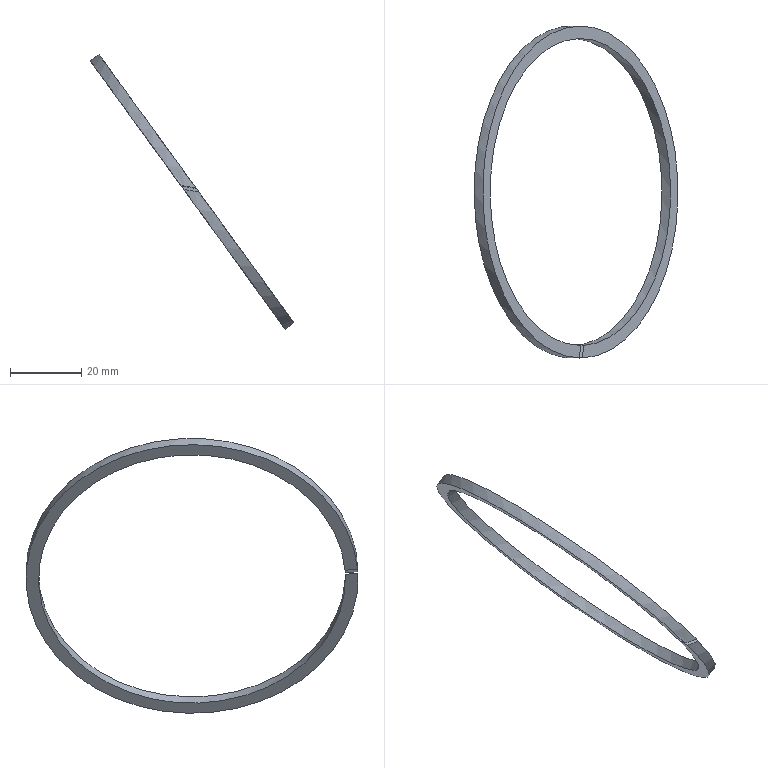Component | NX | PISTON_RING | 1 solid | 6 faces | box 57.09 x 93 x 77 mm | volume 2937 mm3 | plane 4 | cylinder 2 | commonest cylinder face diameters 86 x1 93 x1
STEP:
#1=CARTESIAN_POINT('',(0.,0.,0.));
#2=DIRECTION('',(0.,0.,1.));
#3=DIRECTION('',(1.,0.,0.));
#4=AXIS2_PLACEMENT_3D('',#1,#2,#3);
#5=CARTESIAN_POINT('',(-195.667,-43.,-142.088));
#6=VERTEX_POINT('',#5);
#7=CARTESIAN_POINT('',(-199.858,-42.891,-141.424));
#8=VERTEX_POINT('',#7);
#9=CARTESIAN_POINT('',(-198.06,-0.,-143.899));
#10=DIRECTION('',(-0.1575,-0.0503,-0.9862));
#11=DIRECTION('',(-0.9866,0.0503,0.155));
#12=AXIS2_PLACEMENT_3D('',#9,#10,#11);
#13=ELLIPSE('',#12,60.811,43.);
#14=CARTESIAN_POINT('',(-195.633,-0.,-142.136));
#15=DIRECTION('',(-0.809,0.,-0.5878));
#16=DIRECTION('',(-0.5863,0.07113,0.807));
#17=AXIS2_PLACEMENT_3D('',#14,#15,#16);
#18=CYLINDRICAL_SURFACE('',#17,43.);
#19=CARTESIAN_POINT('',(-1.641,0.));
#20=CARTESIAN_POINT('',(-1.571,3.));
#21=B_SPLINE_CURVE_WITH_KNOTS('',1,(#19,#20),.UNSPECIFIED.,.F.,.F.,(2,2),(4.643,4.712),.PIECEWISE_BEZIER_KNOTS.);
#22=(GEOMETRIC_REPRESENTATION_CONTEXT(2)PARAMETRIC_REPRESENTATION_CONTEXT()REPRESENTATION_CONTEXT('',''));
#23=DEFINITIONAL_REPRESENTATION('',(#21),#22);
#24=PCURVE('',#18,#23);
#25=CARTESIAN_POINT('',(-213.121,-459.397,-118.066));
#26=DIRECTION('',(-0.1575,-0.0503,-0.9862));
#27=DIRECTION('',(-0.9866,0.0503,0.155));
#28=AXIS2_PLACEMENT_3D('',#25,#26,#27);
#29=PLANE('',#28);
#30=CARTESIAN_POINT('',(4.243,460.35));
#31=DIRECTION('',(1.,0.));
#32=AXIS2_PLACEMENT_2D('',#30,#31);
#33=ELLIPSE('',#32,60.811,43.);
#34=(GEOMETRIC_REPRESENTATION_CONTEXT(2)PARAMETRIC_REPRESENTATION_CONTEXT()REPRESENTATION_CONTEXT('',''));
#35=DEFINITIONAL_REPRESENTATION('',(#33),#34);
#36=PCURVE('',#29,#35);
#37=SURFACE_CURVE('',#13,(#24,#36),.PCURVE_S1.);
#38=EDGE_CURVE('',#6,#8,#37,.T.);
#39=ORIENTED_EDGE('',*,*,#38,.F.);
#40=CARTESIAN_POINT('',(-194.833,-42.978,-143.236));
#41=VERTEX_POINT('',#40);
#42=CARTESIAN_POINT('',(-195.633,-0.,-142.136));
#43=DIRECTION('',(0.809,0.,0.5878));
#44=DIRECTION('',(0.5863,-0.07113,-0.807));
#45=AXIS2_PLACEMENT_3D('',#42,#43,#44);
#46=CIRCLE('',#45,43.);
#47=CARTESIAN_POINT('',(9.425,-0.));
#48=DIRECTION('',(-1.,0.));
#49=VECTOR('',#48,1.);
#50=LINE('',#47,#49);
#51=(GEOMETRIC_REPRESENTATION_CONTEXT(2)PARAMETRIC_REPRESENTATION_CONTEXT()REPRESENTATION_CONTEXT('',''));
#52=DEFINITIONAL_REPRESENTATION('',(#50),#51);
#53=PCURVE('',#18,#52);
#54=CARTESIAN_POINT('',(-195.633,-0.,-142.136));
#55=DIRECTION('',(0.809,0.,0.5878));
#56=DIRECTION('',(0.5863,-0.07113,-0.807));
#57=AXIS2_PLACEMENT_3D('',#54,#55,#56);
#58=PLANE('',#57);
#59=CARTESIAN_POINT('',(0.,0.));
#60=DIRECTION('',(1.,0.));
#61=AXIS2_PLACEMENT_2D('',#59,#60);
#62=CIRCLE('',#61,43.);
#63=(GEOMETRIC_REPRESENTATION_CONTEXT(2)PARAMETRIC_REPRESENTATION_CONTEXT()REPRESENTATION_CONTEXT('',''));
#64=DEFINITIONAL_REPRESENTATION('',(#62),#63);
#65=PCURVE('',#58,#64);
#66=SURFACE_CURVE('',#46,(#53,#65),.PCURVE_S1.);
#67=EDGE_CURVE('',#41,#6,#66,.T.);
#68=ORIENTED_EDGE('',*,*,#67,.F.);
#69=CARTESIAN_POINT('',(-199.027,-42.968,-142.567));
#70=VERTEX_POINT('',#69);
#71=CARTESIAN_POINT('',(-199.204,-0.,-144.73));
#72=DIRECTION('',(0.1575,0.0503,0.9862));
#73=DIRECTION('',(-0.9866,0.0503,0.155));
#74=AXIS2_PLACEMENT_3D('',#71,#72,#73);
#75=ELLIPSE('',#74,60.811,43.);
#76=CARTESIAN_POINT('',(4.679,3.));
#77=CARTESIAN_POINT('',(4.61,0.));
#78=B_SPLINE_CURVE_WITH_KNOTS('',1,(#76,#77),.UNSPECIFIED.,.F.,.F.,(2,2),(1.604,1.674),.PIECEWISE_BEZIER_KNOTS.);
#79=(GEOMETRIC_REPRESENTATION_CONTEXT(2)PARAMETRIC_REPRESENTATION_CONTEXT()REPRESENTATION_CONTEXT('',''));
#80=DEFINITIONAL_REPRESENTATION('',(#78),#79);
#81=PCURVE('',#18,#80);
#82=CARTESIAN_POINT('',(-216.477,-459.285,-118.549));
#83=DIRECTION('',(0.1575,0.0503,0.9862));
#84=DIRECTION('',(0.9866,-0.0503,-0.155));
#85=AXIS2_PLACEMENT_3D('',#82,#83,#84);
#86=PLANE('',#85);
#87=CARTESIAN_POINT('',(-2.,460.35));
#88=DIRECTION('',(-1.,0.));
#89=AXIS2_PLACEMENT_2D('',#87,#88);
#90=ELLIPSE('',#89,60.811,43.);
#91=(GEOMETRIC_REPRESENTATION_CONTEXT(2)PARAMETRIC_REPRESENTATION_CONTEXT()REPRESENTATION_CONTEXT('',''));
#92=DEFINITIONAL_REPRESENTATION('',(#90),#91);
#93=PCURVE('',#86,#92);
#94=SURFACE_CURVE('',#75,(#81,#93),.PCURVE_S1.);
#95=EDGE_CURVE('',#70,#41,#94,.T.);
#96=ORIENTED_EDGE('',*,*,#95,.F.);
#97=CARTESIAN_POINT('',(-198.06,-0.,-143.899));
#98=DIRECTION('',(0.809,0.,0.5878));
#99=DIRECTION('',(0.5863,-0.07113,-0.807));
#100=AXIS2_PLACEMENT_3D('',#97,#98,#99);
#101=CIRCLE('',#100,43.);
#102=CARTESIAN_POINT('',(9.425,3.));
#103=DIRECTION('',(-1.,0.));
#104=VECTOR('',#103,1.);
#105=LINE('',#102,#104);
#106=(GEOMETRIC_REPRESENTATION_CONTEXT(2)PARAMETRIC_REPRESENTATION_CONTEXT()REPRESENTATION_CONTEXT('',''));
#107=DEFINITIONAL_REPRESENTATION('',(#105),#106);
#108=PCURVE('',#18,#107);
#109=CARTESIAN_POINT('',(-198.06,-0.,-143.899));
#110=DIRECTION('',(0.809,0.,0.5878));
#111=DIRECTION('',(0.5863,-0.07113,-0.807));
#112=AXIS2_PLACEMENT_3D('',#109,#110,#111);
#113=PLANE('',#112);
#114=CARTESIAN_POINT('',(0.,0.));
#115=DIRECTION('',(1.,0.));
#116=AXIS2_PLACEMENT_2D('',#114,#115);
#117=CIRCLE('',#116,43.);
#118=(GEOMETRIC_REPRESENTATION_CONTEXT(2)PARAMETRIC_REPRESENTATION_CONTEXT()REPRESENTATION_CONTEXT('',''));
#119=DEFINITIONAL_REPRESENTATION('',(#117),#118);
#120=PCURVE('',#113,#119);
#121=SURFACE_CURVE('',#101,(#108,#120),.PCURVE_S1.);
#122=EDGE_CURVE('',#70,#8,#121,.T.);
#123=ORIENTED_EDGE('',*,*,#122,.T.);
#124=EDGE_LOOP('',(#39,#68,#96,#123));
#125=FACE_BOUND('',#124,.F.);
#126=ADVANCED_FACE('',(#125),#18,.F.);
#127=CARTESIAN_POINT('',(-194.98,-46.487,-143.034));
#128=VERTEX_POINT('',#127);
#129=CARTESIAN_POINT('',(-195.814,-46.499,-141.886));
#130=VERTEX_POINT('',#129);
#131=CARTESIAN_POINT('',(-195.633,-0.,-142.136));
#132=DIRECTION('',(0.809,0.,0.5878));
#133=DIRECTION('',(0.5863,-0.07113,-0.807));
#134=AXIS2_PLACEMENT_3D('',#131,#132,#133);
#135=CIRCLE('',#134,46.5);
#136=CARTESIAN_POINT('',(0.,0.));
#137=DIRECTION('',(1.,0.));
#138=AXIS2_PLACEMENT_2D('',#136,#137);
#139=CIRCLE('',#138,46.5);
#140=(GEOMETRIC_REPRESENTATION_CONTEXT(2)PARAMETRIC_REPRESENTATION_CONTEXT()REPRESENTATION_CONTEXT('',''));
#141=DEFINITIONAL_REPRESENTATION('',(#139),#140);
#142=PCURVE('',#58,#141);
#143=CARTESIAN_POINT('',(-195.633,-0.,-142.136));
#144=DIRECTION('',(-0.809,0.,-0.5878));
#145=DIRECTION('',(-0.5863,0.07113,0.807));
#146=AXIS2_PLACEMENT_3D('',#143,#144,#145);
#147=CYLINDRICAL_SURFACE('',#146,46.5);
#148=CARTESIAN_POINT('',(9.425,-0.));
#149=DIRECTION('',(-1.,0.));
#150=VECTOR('',#149,1.);
#151=LINE('',#148,#150);
#152=(GEOMETRIC_REPRESENTATION_CONTEXT(2)PARAMETRIC_REPRESENTATION_CONTEXT()REPRESENTATION_CONTEXT('',''));
#153=DEFINITIONAL_REPRESENTATION('',(#151),#152);
#154=PCURVE('',#147,#153);
#155=SURFACE_CURVE('',#135,(#142,#154),.PCURVE_S1.);
#156=EDGE_CURVE('',#128,#130,#155,.T.);
#157=ORIENTED_EDGE('',*,*,#156,.T.);
#158=CARTESIAN_POINT('',(-213.121,-459.397,-118.066));
#159=DIRECTION('',(0.04181,0.9975,-0.05754));
#160=VECTOR('',#159,1.);
#161=LINE('',#158,#160);
#162=CARTESIAN_POINT('',(3.,-460.35));
#163=DIRECTION('',(0.,1.));
#164=VECTOR('',#163,1.);
#165=LINE('',#162,#164);
#166=(GEOMETRIC_REPRESENTATION_CONTEXT(2)PARAMETRIC_REPRESENTATION_CONTEXT()REPRESENTATION_CONTEXT('',''));
#167=DEFINITIONAL_REPRESENTATION('',(#165),#166);
#168=PCURVE('',#58,#167);
#169=CARTESIAN_POINT('',(0.,0.));
#170=DIRECTION('',(-0.,1.));
#171=VECTOR('',#170,1.);
#172=LINE('',#169,#171);
#173=(GEOMETRIC_REPRESENTATION_CONTEXT(2)PARAMETRIC_REPRESENTATION_CONTEXT()REPRESENTATION_CONTEXT('',''));
#174=DEFINITIONAL_REPRESENTATION('',(#172),#173);
#175=PCURVE('',#29,#174);
#176=SURFACE_CURVE('',#161,(#168,#175),.PCURVE_S1.);
#177=EDGE_CURVE('',#130,#6,#176,.T.);
#178=ORIENTED_EDGE('',*,*,#177,.T.);
#179=ORIENTED_EDGE('',*,*,#67,.F.);
#180=CARTESIAN_POINT('',(-212.291,-459.498,-119.207));
#181=DIRECTION('',(0.04181,0.9975,-0.05754));
#182=VECTOR('',#181,1.);
#183=LINE('',#180,#182);
#184=CARTESIAN_POINT('',(4.414,-460.35));
#185=DIRECTION('',(0.,1.));
#186=VECTOR('',#185,1.);
#187=LINE('',#184,#186);
#188=(GEOMETRIC_REPRESENTATION_CONTEXT(2)PARAMETRIC_REPRESENTATION_CONTEXT()REPRESENTATION_CONTEXT('',''));
#189=DEFINITIONAL_REPRESENTATION('',(#187),#188);
#190=PCURVE('',#58,#189);
#191=CARTESIAN_POINT('',(4.243,0.));
#192=DIRECTION('',(0.,1.));
#193=VECTOR('',#192,1.);
#194=LINE('',#191,#193);
#195=(GEOMETRIC_REPRESENTATION_CONTEXT(2)PARAMETRIC_REPRESENTATION_CONTEXT()REPRESENTATION_CONTEXT('',''));
#196=DEFINITIONAL_REPRESENTATION('',(#194),#195);
#197=PCURVE('',#86,#196);
#198=SURFACE_CURVE('',#183,(#190,#197),.PCURVE_S1.);
#199=EDGE_CURVE('',#128,#41,#198,.T.);
#200=ORIENTED_EDGE('',*,*,#199,.F.);
#201=EDGE_LOOP('',(#157,#178,#179,#200));
#202=FACE_BOUND('',#201,.T.);
#203=ADVANCED_FACE('',(#202),#58,.T.);
#204=ORIENTED_EDGE('',*,*,#156,.F.);
#205=CARTESIAN_POINT('',(-199.174,-46.461,-142.366));
#206=VERTEX_POINT('',#205);
#207=CARTESIAN_POINT('',(-199.204,-0.,-144.73));
#208=DIRECTION('',(-0.1575,-0.0503,-0.9862));
#209=DIRECTION('',(-0.9866,0.0503,0.155));
#210=AXIS2_PLACEMENT_3D('',#207,#208,#209);
#211=ELLIPSE('',#210,65.761,46.5);
#212=CARTESIAN_POINT('',(4.617,0.));
#213=CARTESIAN_POINT('',(4.682,3.));
#214=B_SPLINE_CURVE_WITH_KNOTS('',1,(#212,#213),.UNSPECIFIED.,.F.,.F.,(2,2),(4.617,4.682),.PIECEWISE_BEZIER_KNOTS.);
#215=(GEOMETRIC_REPRESENTATION_CONTEXT(2)PARAMETRIC_REPRESENTATION_CONTEXT()REPRESENTATION_CONTEXT('',''));
#216=DEFINITIONAL_REPRESENTATION('',(#214),#215);
#217=PCURVE('',#147,#216);
#218=CARTESIAN_POINT('',(-67.761,460.35));
#219=CARTESIAN_POINT('',(-67.761,540.89));
#220=CARTESIAN_POINT('',(30.88,500.62));
#221=CARTESIAN_POINT('',(129.522,460.35));
#222=CARTESIAN_POINT('',(30.88,420.08));
#223=CARTESIAN_POINT('',(-67.761,379.81));
#224=CARTESIAN_POINT('',(-67.761,460.35));
#225=(BOUNDED_CURVE()B_SPLINE_CURVE(2,(#218,#219,#220,#221,#222,#223,#224),.UNSPECIFIED.,.T.,.F.)B_SPLINE_CURVE_WITH_KNOTS((1,2,2,2,2,1),(-2.094,0.,2.094,4.189,6.283,8.378),.UNSPECIFIED.)CURVE()GEOMETRIC_REPRESENTATION_ITEM()RATIONAL_B_SPLINE_CURVE((1.,0.5,1.,0.5,1.,0.5,1.))REPRESENTATION_ITEM(''));
#226=(GEOMETRIC_REPRESENTATION_CONTEXT(2)PARAMETRIC_REPRESENTATION_CONTEXT()REPRESENTATION_CONTEXT('',''));
#227=DEFINITIONAL_REPRESENTATION('',(#225),#226);
#228=PCURVE('',#86,#227);
#229=SURFACE_CURVE('',#211,(#217,#228),.PCURVE_S1.);
#230=EDGE_CURVE('',#128,#206,#229,.T.);
#231=ORIENTED_EDGE('',*,*,#230,.T.);
#232=CARTESIAN_POINT('',(-200.004,-46.382,-141.223));
#233=VERTEX_POINT('',#232);
#234=CARTESIAN_POINT('',(-198.06,-0.,-143.899));
#235=DIRECTION('',(0.809,0.,0.5878));
#236=DIRECTION('',(0.5863,-0.07113,-0.807));
#237=AXIS2_PLACEMENT_3D('',#234,#235,#236);
#238=CIRCLE('',#237,46.5);
#239=CARTESIAN_POINT('',(9.425,3.));
#240=DIRECTION('',(-1.,0.));
#241=VECTOR('',#240,1.);
#242=LINE('',#239,#241);
#243=(GEOMETRIC_REPRESENTATION_CONTEXT(2)PARAMETRIC_REPRESENTATION_CONTEXT()REPRESENTATION_CONTEXT('',''));
#244=DEFINITIONAL_REPRESENTATION('',(#242),#243);
#245=PCURVE('',#147,#244);
#246=CARTESIAN_POINT('',(0.,0.));
#247=DIRECTION('',(1.,0.));
#248=AXIS2_PLACEMENT_2D('',#246,#247);
#249=CIRCLE('',#248,46.5);
#250=(GEOMETRIC_REPRESENTATION_CONTEXT(2)PARAMETRIC_REPRESENTATION_CONTEXT()REPRESENTATION_CONTEXT('',''));
#251=DEFINITIONAL_REPRESENTATION('',(#249),#250);
#252=PCURVE('',#113,#251);
#253=SURFACE_CURVE('',#238,(#245,#252),.PCURVE_S1.);
#254=EDGE_CURVE('',#206,#233,#253,.T.);
#255=ORIENTED_EDGE('',*,*,#254,.T.);
#256=CARTESIAN_POINT('',(-198.06,-0.,-143.899));
#257=DIRECTION('',(0.1575,0.0503,0.9862));
#258=DIRECTION('',(-0.9866,0.0503,0.155));
#259=AXIS2_PLACEMENT_3D('',#256,#257,#258);
#260=ELLIPSE('',#259,65.761,46.5);
#261=CARTESIAN_POINT('',(-1.571,3.));
#262=CARTESIAN_POINT('',(-1.635,0.));
#263=B_SPLINE_CURVE_WITH_KNOTS('',1,(#261,#262),.UNSPECIFIED.,.F.,.F.,(2,2),(1.571,1.635),.PIECEWISE_BEZIER_KNOTS.);
#264=(GEOMETRIC_REPRESENTATION_CONTEXT(2)PARAMETRIC_REPRESENTATION_CONTEXT()REPRESENTATION_CONTEXT('',''));
#265=DEFINITIONAL_REPRESENTATION('',(#263),#264);
#266=PCURVE('',#147,#265);
#267=CARTESIAN_POINT('',(70.004,460.35));
#268=CARTESIAN_POINT('',(70.004,379.81));
#269=CARTESIAN_POINT('',(-28.638,420.08));
#270=CARTESIAN_POINT('',(-127.279,460.35));
#271=CARTESIAN_POINT('',(-28.638,500.62));
#272=CARTESIAN_POINT('',(70.004,540.89));
#273=CARTESIAN_POINT('',(70.004,460.35));
#274=(BOUNDED_CURVE()B_SPLINE_CURVE(2,(#267,#268,#269,#270,#271,#272,#273),.UNSPECIFIED.,.T.,.F.)B_SPLINE_CURVE_WITH_KNOTS((1,2,2,2,2,1),(-2.094,0.,2.094,4.189,6.283,8.378),.UNSPECIFIED.)CURVE()GEOMETRIC_REPRESENTATION_ITEM()RATIONAL_B_SPLINE_CURVE((1.,0.5,1.,0.5,1.,0.5,1.))REPRESENTATION_ITEM(''));
#275=(GEOMETRIC_REPRESENTATION_CONTEXT(2)PARAMETRIC_REPRESENTATION_CONTEXT()REPRESENTATION_CONTEXT('',''));
#276=DEFINITIONAL_REPRESENTATION('',(#274),#275);
#277=PCURVE('',#29,#276);
#278=SURFACE_CURVE('',#260,(#266,#277),.PCURVE_S1.);
#279=EDGE_CURVE('',#233,#130,#278,.T.);
#280=ORIENTED_EDGE('',*,*,#279,.T.);
#281=EDGE_LOOP('',(#204,#231,#255,#280));
#282=FACE_BOUND('',#281,.T.);
#283=ADVANCED_FACE('',(#282),#147,.T.);
#284=ORIENTED_EDGE('',*,*,#254,.F.);
#285=CARTESIAN_POINT('',(-216.477,-459.285,-118.549));
#286=DIRECTION('',(0.04181,0.9975,-0.05754));
#287=VECTOR('',#286,1.);
#288=LINE('',#285,#287);
#289=CARTESIAN_POINT('',(1.414,-460.35));
#290=DIRECTION('',(0.,1.));
#291=VECTOR('',#290,1.);
#292=LINE('',#289,#291);
#293=(GEOMETRIC_REPRESENTATION_CONTEXT(2)PARAMETRIC_REPRESENTATION_CONTEXT()REPRESENTATION_CONTEXT('',''));
#294=DEFINITIONAL_REPRESENTATION('',(#292),#293);
#295=PCURVE('',#113,#294);
#296=CARTESIAN_POINT('',(0.,0.));
#297=DIRECTION('',(0.,1.));
#298=VECTOR('',#297,1.);
#299=LINE('',#296,#298);
#300=(GEOMETRIC_REPRESENTATION_CONTEXT(2)PARAMETRIC_REPRESENTATION_CONTEXT()REPRESENTATION_CONTEXT('',''));
#301=DEFINITIONAL_REPRESENTATION('',(#299),#300);
#302=PCURVE('',#86,#301);
#303=SURFACE_CURVE('',#288,(#295,#302),.PCURVE_S1.);
#304=EDGE_CURVE('',#206,#70,#303,.T.);
#305=ORIENTED_EDGE('',*,*,#304,.T.);
#306=ORIENTED_EDGE('',*,*,#122,.T.);
#307=CARTESIAN_POINT('',(-217.307,-459.184,-117.408));
#308=DIRECTION('',(0.04181,0.9975,-0.05754));
#309=VECTOR('',#308,1.);
#310=LINE('',#307,#309);
#311=CARTESIAN_POINT('',(-0.,-460.35));
#312=DIRECTION('',(0.,1.));
#313=VECTOR('',#312,1.);
#314=LINE('',#311,#313);
#315=(GEOMETRIC_REPRESENTATION_CONTEXT(2)PARAMETRIC_REPRESENTATION_CONTEXT()REPRESENTATION_CONTEXT('',''));
#316=DEFINITIONAL_REPRESENTATION('',(#314),#315);
#317=PCURVE('',#113,#316);
#318=CARTESIAN_POINT('',(4.243,0.));
#319=DIRECTION('',(-0.,1.));
#320=VECTOR('',#319,1.);
#321=LINE('',#318,#320);
#322=(GEOMETRIC_REPRESENTATION_CONTEXT(2)PARAMETRIC_REPRESENTATION_CONTEXT()REPRESENTATION_CONTEXT('',''));
#323=DEFINITIONAL_REPRESENTATION('',(#321),#322);
#324=PCURVE('',#29,#323);
#325=SURFACE_CURVE('',#310,(#317,#324),.PCURVE_S1.);
#326=EDGE_CURVE('',#233,#8,#325,.T.);
#327=ORIENTED_EDGE('',*,*,#326,.F.);
#328=EDGE_LOOP('',(#284,#305,#306,#327));
#329=FACE_BOUND('',#328,.T.);
#330=ADVANCED_FACE('',(#329),#113,.F.);
#331=ORIENTED_EDGE('',*,*,#177,.F.);
#332=ORIENTED_EDGE('',*,*,#279,.F.);
#333=ORIENTED_EDGE('',*,*,#326,.T.);
#334=ORIENTED_EDGE('',*,*,#38,.F.);
#335=EDGE_LOOP('',(#331,#332,#333,#334));
#336=FACE_BOUND('',#335,.T.);
#337=ADVANCED_FACE('',(#336),#29,.T.);
#338=ORIENTED_EDGE('',*,*,#304,.F.);
#339=ORIENTED_EDGE('',*,*,#230,.F.);
#340=ORIENTED_EDGE('',*,*,#199,.T.);
#341=ORIENTED_EDGE('',*,*,#95,.F.);
#342=EDGE_LOOP('',(#338,#339,#340,#341));
#343=FACE_BOUND('',#342,.T.);
#344=ADVANCED_FACE('',(#343),#86,.T.);
#345=CLOSED_SHELL('',(#126,#203,#283,#330,#337,#344));
#346=MANIFOLD_SOLID_BREP('',#345);
#347=(LENGTH_UNIT()NAMED_UNIT(*)SI_UNIT(.MILLI.,.METRE.));
#348=UNCERTAINTY_MEASURE_WITH_UNIT(LENGTH_MEASURE(0.001),#347,'','');
#349=(NAMED_UNIT(*)PLANE_ANGLE_UNIT()SI_UNIT($,.RADIAN.));
#350=(NAMED_UNIT(*)SI_UNIT($,.STERADIAN.)SOLID_ANGLE_UNIT());
#351=(GEOMETRIC_REPRESENTATION_CONTEXT(3)GLOBAL_UNCERTAINTY_ASSIGNED_CONTEXT((#348))GLOBAL_UNIT_ASSIGNED_CONTEXT((#347,#349,#350))REPRESENTATION_CONTEXT('',''));
#352=ADVANCED_BREP_SHAPE_REPRESENTATION('',(#4,#346),#351);